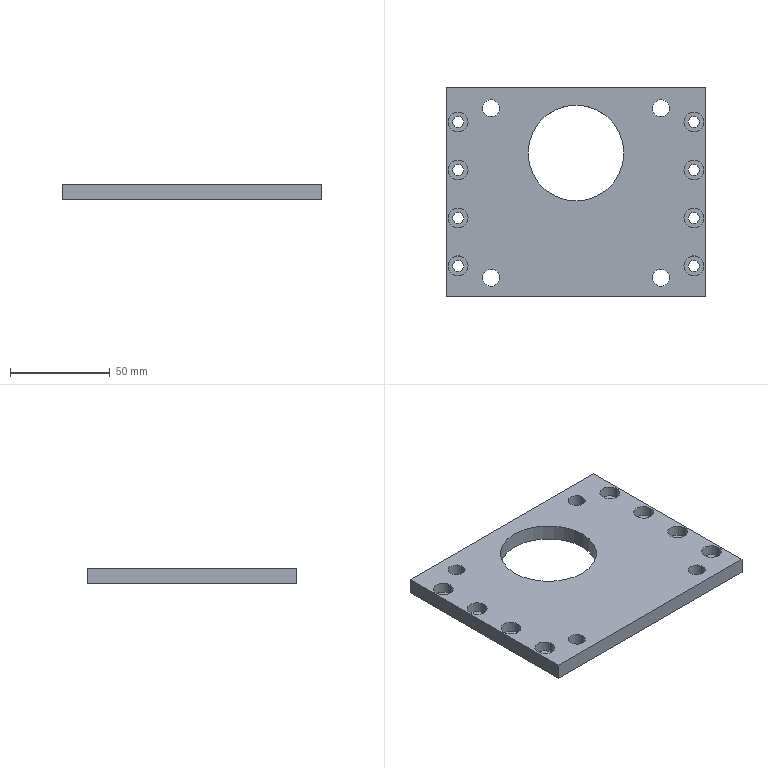Component | SolidWorks | DC-024-06-1 | 1 solid | 56 faces | box 130 x 105 x 8 mm | volume 89021 mm3 | cylinder 42 | plane 14 | commonest cylinder face diameters 10 x16 5.5 x16 8.5 x8 48 x2
build123d program:
from build123d import *

# Parameters (mm, degrees)
SKETCH1_W                                       = 130
SKETCH1_H                                       = 105
BOSS_EXTRUDE1_DEPTH                             = 4
M5_HEX_SOCKET_HEAD_CAP_SCREW_CBORE1_D           = 5.5
M5_HEX_SOCKET_HEAD_CAP_SCREW_CBORE1_DEPTH       = 12.4
M5_HEX_SOCKET_HEAD_CAP_SCREW_CBORE1_CBORE_D     = 10
M5_HEX_SOCKET_HEAD_CAP_SCREW_CBORE1_CBORE_DEPTH = 5.4
M5_HEX_SOCKET_HEAD_CAP_SCREW_CBORE1_TIP         = 1.652
SKETCH5_R                                       = 24
CUT_EXTRUDE1_DEPTH                              = 90.5
F_8_5_8_5_DIAMETER_HOLE1_D                      = 8.5


with BuildPart() as part:
    # Sketch1 → Boss-Extrude1 (new, symmetric)
    with BuildSketch(Plane.XY):
        Rectangle(SKETCH1_W, SKETCH1_H)
    extrude(amount=BOSS_EXTRUDE1_DEPTH, both=True)

    # M5 Hex Socket Head Cap Screw CBORE1
    with Locations(Plane.XY.offset(4)):
        with Locations((59, 35), (59, 11), (59, -13), (59, -37), (-59, -37), (-59, -13), (-59, 11), (-59, 35)):
            CounterBoreHole(M5_HEX_SOCKET_HEAD_CAP_SCREW_CBORE1_D / 2, M5_HEX_SOCKET_HEAD_CAP_SCREW_CBORE1_CBORE_D / 2, M5_HEX_SOCKET_HEAD_CAP_SCREW_CBORE1_CBORE_DEPTH, depth=M5_HEX_SOCKET_HEAD_CAP_SCREW_CBORE1_DEPTH)
            with Locations((0, 0, -(M5_HEX_SOCKET_HEAD_CAP_SCREW_CBORE1_DEPTH + M5_HEX_SOCKET_HEAD_CAP_SCREW_CBORE1_TIP / 2))):  # 118° drill point
                Cone(0, M5_HEX_SOCKET_HEAD_CAP_SCREW_CBORE1_D / 2, M5_HEX_SOCKET_HEAD_CAP_SCREW_CBORE1_TIP, mode=Mode.SUBTRACT)

    # Sketch5 → Cut-Extrude1 (cut)
    with BuildSketch(Plane(origin=(0, 0, -4), x_dir=(-1, 0, 0), z_dir=(0, 0, -1))):
        with Locations((0, 19.5)):
            Circle(SKETCH5_R)
    extrude(amount=-CUT_EXTRUDE1_DEPTH, mode=Mode.SUBTRACT)

    # 8.5 _8.5_ Diameter Hole1 (through all)
    with Locations(Plane.XY.offset(4)):
        with Locations((-42.5, 42), (42.5, 42), (-42.5, -43), (42.5, -43)):
            Hole(F_8_5_8_5_DIAMETER_HOLE1_D / 2)


solid = part.part

# Placed as in the assembly
solid = solid.moved(Location((-25.633, -394.091, 57), (0, 0, 0)))